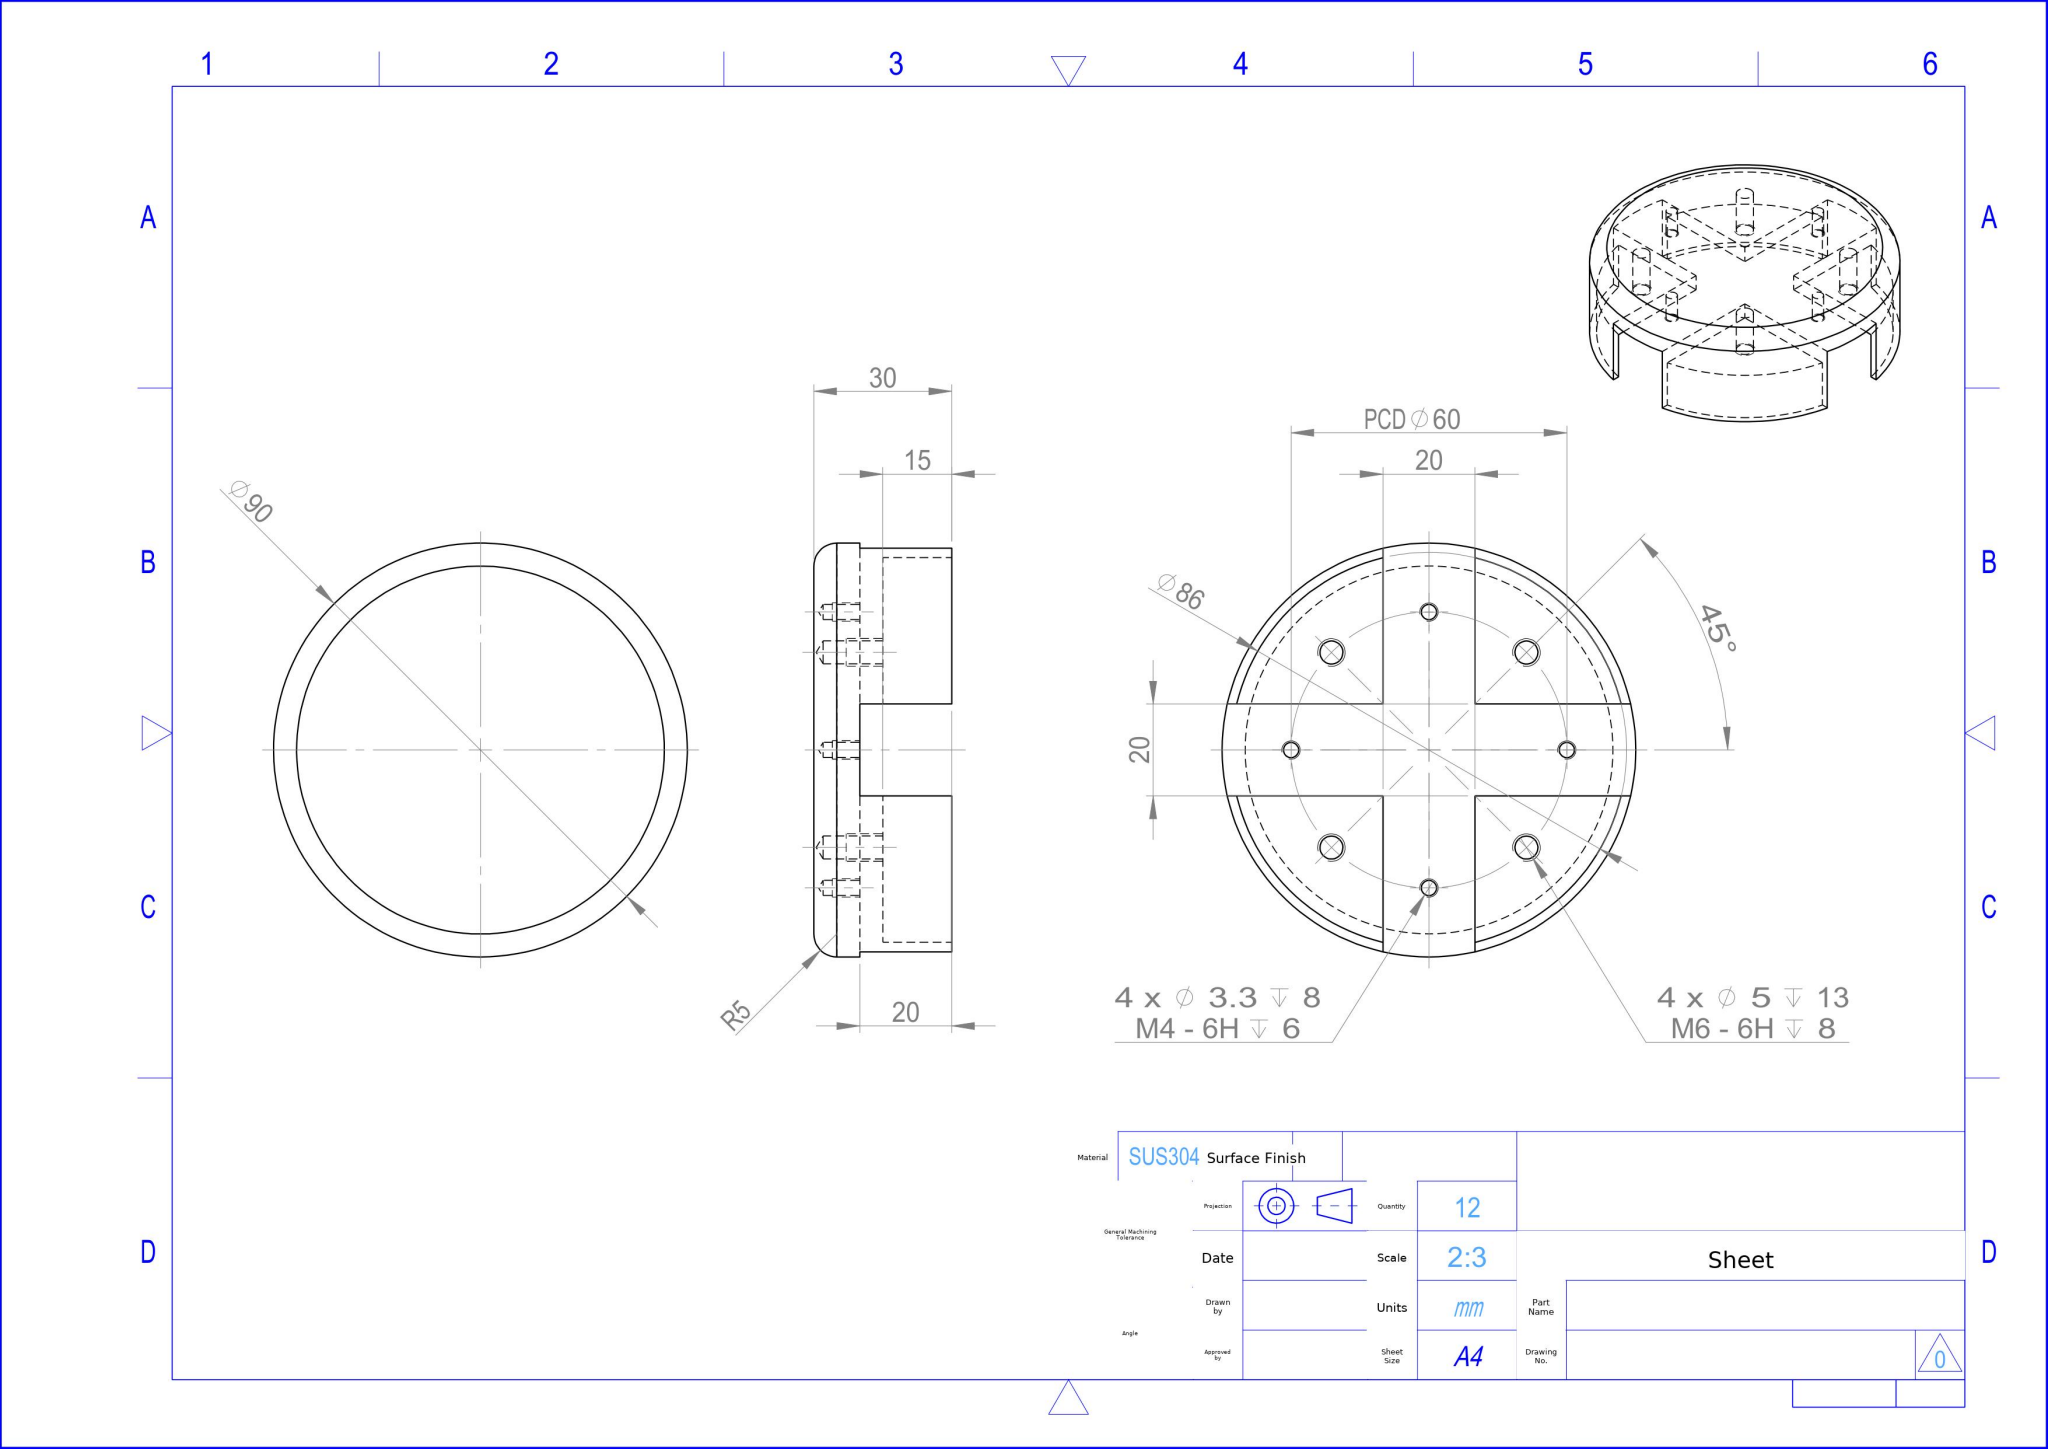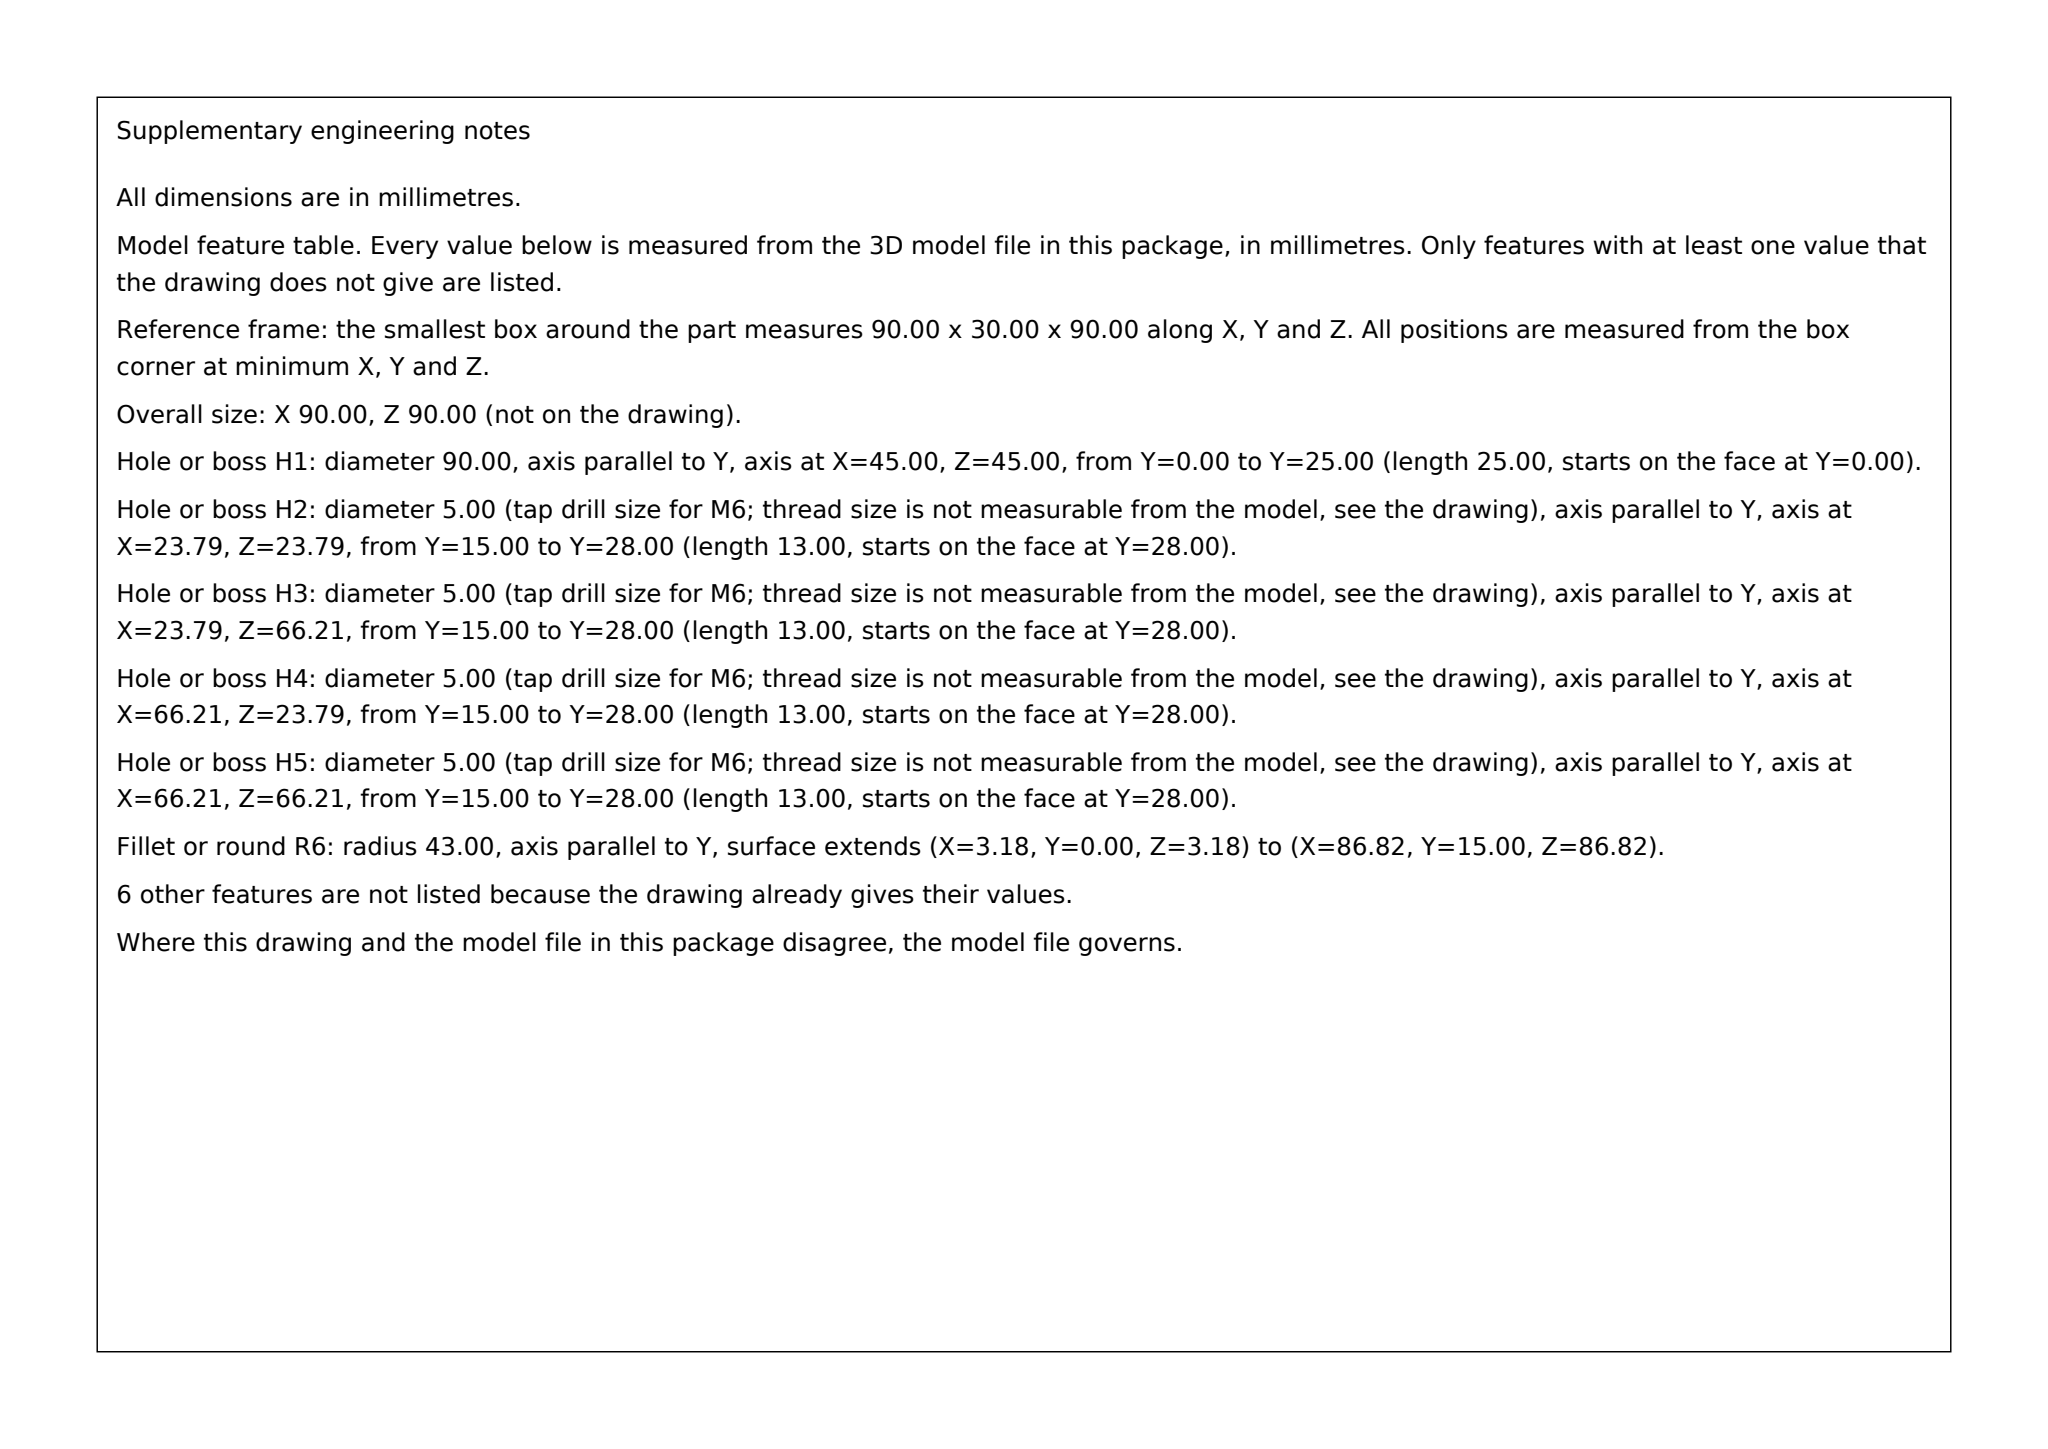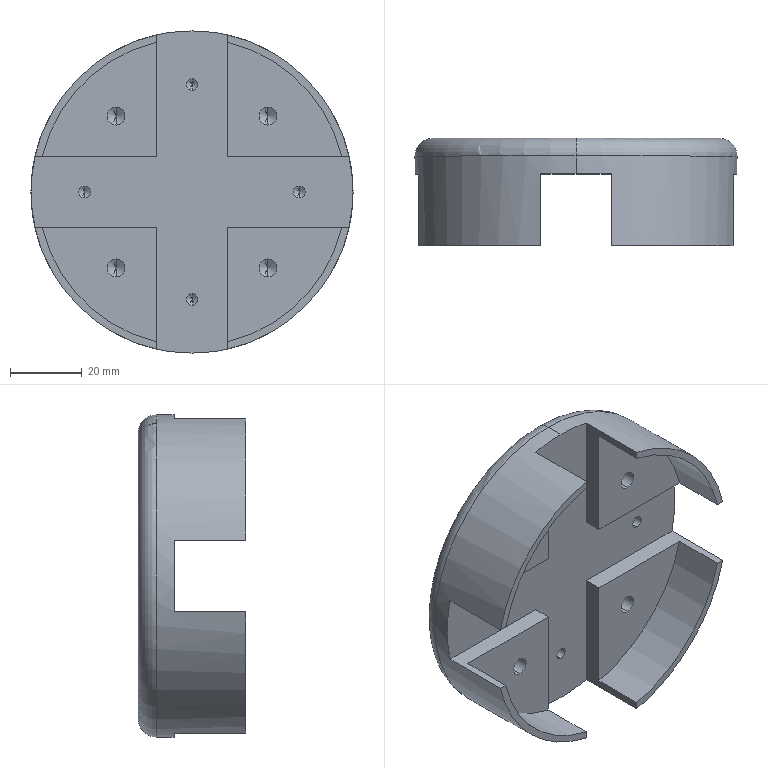Part | SolidWorks | mm | material SUS304 | 1 solid | 58 faces | box 90 x 30 x 90 mm | volume 82623 mm3 | cylinder 22 | plane 18 | cone 16 | torus 2 | commonest cylinder face diameters 3.3 x8 5 x8 86 x4 90 x2
build123d program:
from build123d import *

# Parameters (mm, degrees)
SKETCH1_R             = 45
BOSS_EXTRUDE1_DEPTH   = 30
SKETCH2_R             = 43
CUT_EXTRUDE1_DEPTH    = 15
CUT_EXTRUDE2_DEPTH    = 20
FILLET1_R             = 5
M6_TAPPED_HOLE1_D     = 5
M6_TAPPED_HOLE1_DEPTH = 13
M6_TAPPED_HOLE1_TIP   = 1.502
M4_TAPPED_HOLE1_D     = 3.3
M4_TAPPED_HOLE1_DEPTH = 8
M4_TAPPED_HOLE1_TIP   = 0.9914


with BuildPart() as part:
    # Sketch1 → Boss-Extrude1 (new body)
    with BuildSketch(Plane(origin=(0, 0, 0), x_dir=(1, 0, 0), z_dir=(0, 1, 0))):
        with Locations(Location((0, 0, 0), (0, 0, 270))):
            Circle(SKETCH1_R)
    extrude(amount=BOSS_EXTRUDE1_DEPTH)

    # Sketch2 → Cut-Extrude1 (cut)
    with BuildSketch(Plane(origin=(0, 0, 0), x_dir=(-1, 0, 0), z_dir=(0, -1, 0))):
        with Locations(Location((0, 0, 0), (0, 0, 90))):
            Circle(SKETCH2_R)
    extrude(amount=-CUT_EXTRUDE1_DEPTH, mode=Mode.SUBTRACT)

    # Sketch3 → Cut-Extrude2 (cut)
    with BuildSketch(Plane.XZ):
        Polygon((-47.5, 10), (-10, 10), (-10, 47.5), (10, 47.5), (10, 10), (47.5, 10), (47.5, -10), (10, -10), (10, -47.5), (-10, -47.5), (-10, -10), (-47.5, -10), align=None)
    extrude(amount=-CUT_EXTRUDE2_DEPTH, mode=Mode.SUBTRACT)

    # Fillet1
    fillet1_edges = [part.edges().sort_by_distance(p)[0] for p in [
        (0, 30, -45),
    ]]
    fillet(fillet1_edges, radius=FILLET1_R)

    # M6 Tapped Hole1
    with Locations(Plane(origin=(0, 15, 0), x_dir=(-1, 0, 0), z_dir=(0, -1, 0))):
        with Locations((21.213, -21.213), (-21.213, 21.213), (-21.213, -21.213), (21.213, 21.213)):
            Hole(M6_TAPPED_HOLE1_D / 2, depth=M6_TAPPED_HOLE1_DEPTH)
            with Locations((0, 0, -(M6_TAPPED_HOLE1_DEPTH + M6_TAPPED_HOLE1_TIP / 2))):  # 118° drill point
                Cone(0, M6_TAPPED_HOLE1_D / 2, M6_TAPPED_HOLE1_TIP, mode=Mode.SUBTRACT)

    # M4 Tapped Hole1
    with Locations(Plane(origin=(0, 20, 0), x_dir=(-1, 0, 0), z_dir=(0, -1, 0))):
        with Locations((0, -30), (0, 30), (30, 0), (-30, 0)):
            Hole(M4_TAPPED_HOLE1_D / 2, depth=M4_TAPPED_HOLE1_DEPTH)
            with Locations((0, 0, -(M4_TAPPED_HOLE1_DEPTH + M4_TAPPED_HOLE1_TIP / 2))):  # 118° drill point
                Cone(0, M4_TAPPED_HOLE1_D / 2, M4_TAPPED_HOLE1_TIP, mode=Mode.SUBTRACT)


solid = part.part